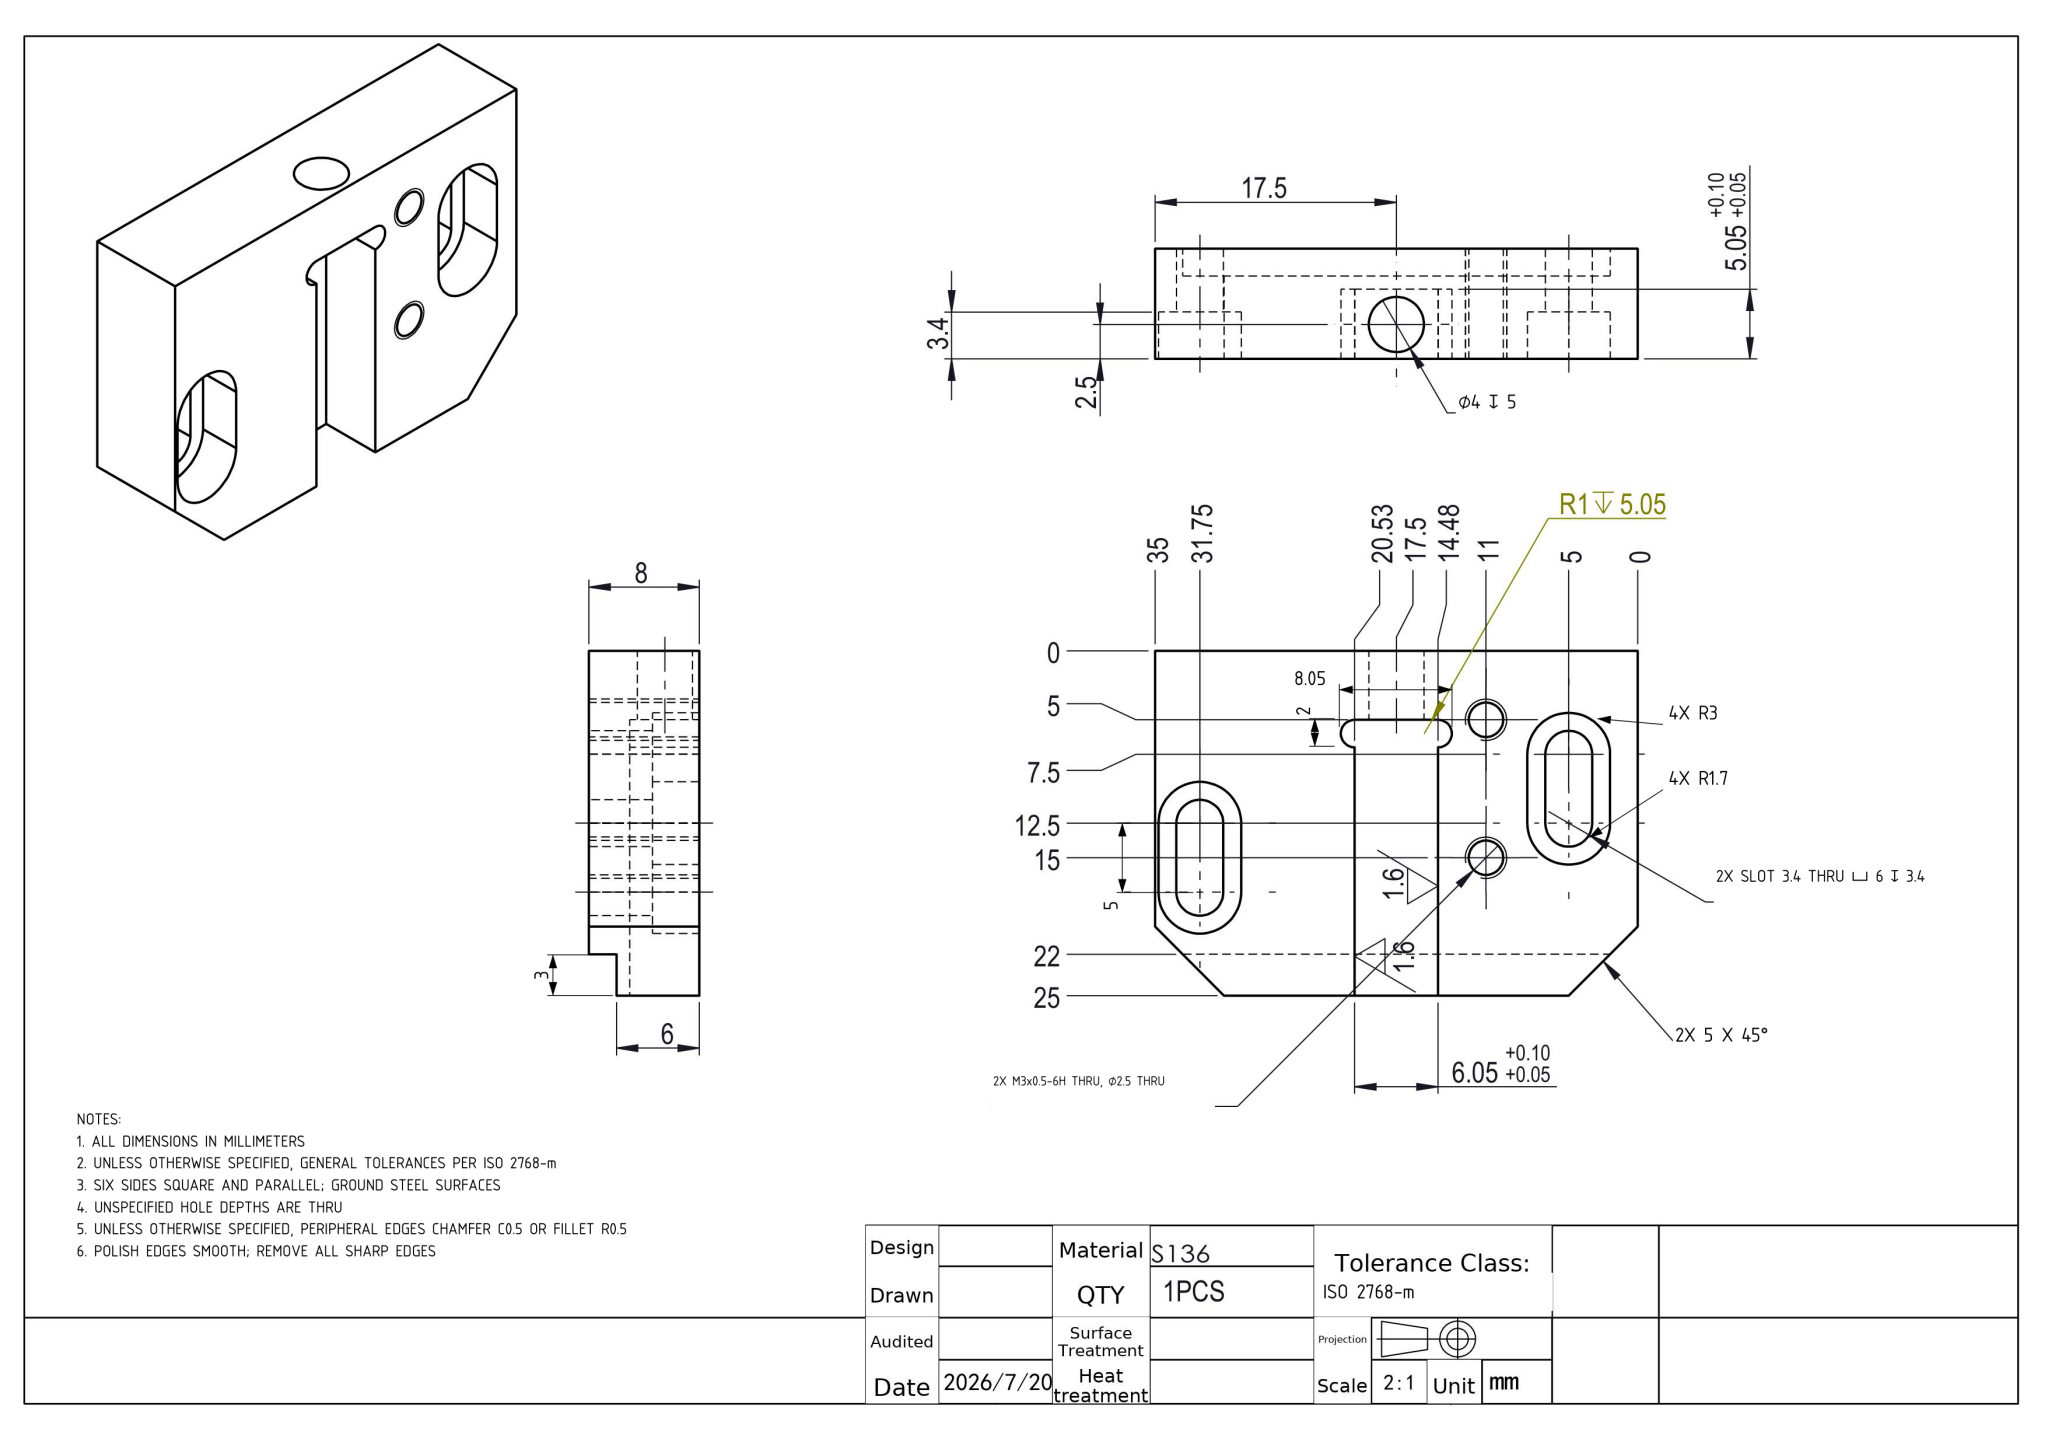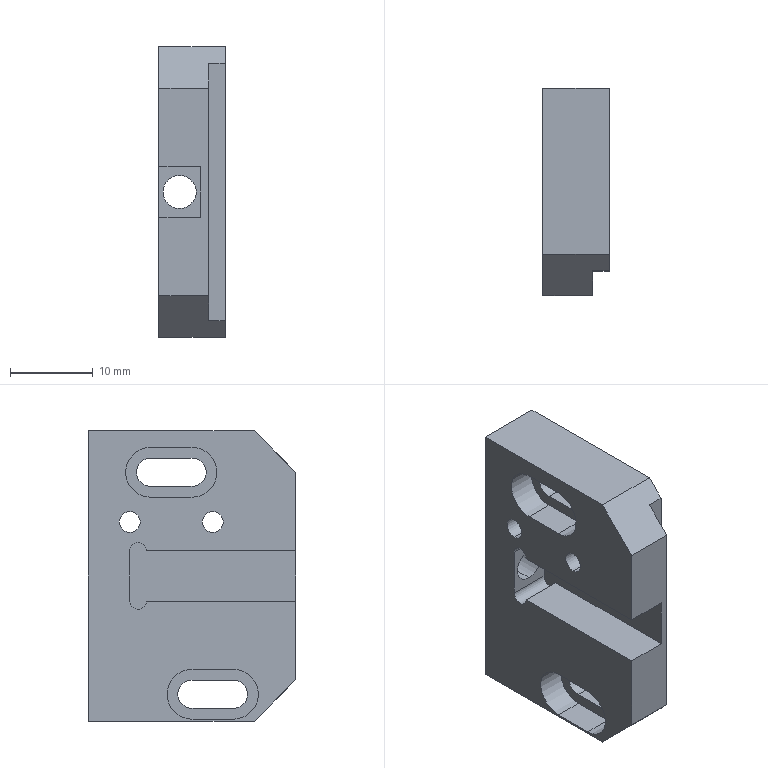Part | NX | mm | 1 solid | 41 faces | box 8 x 25 x 35 mm | volume 5228 mm3 | plane 24 | cylinder 17 | commonest cylinder face diameters 2.5 x4 6 x4 3.4 x4 2 x3 4 x2